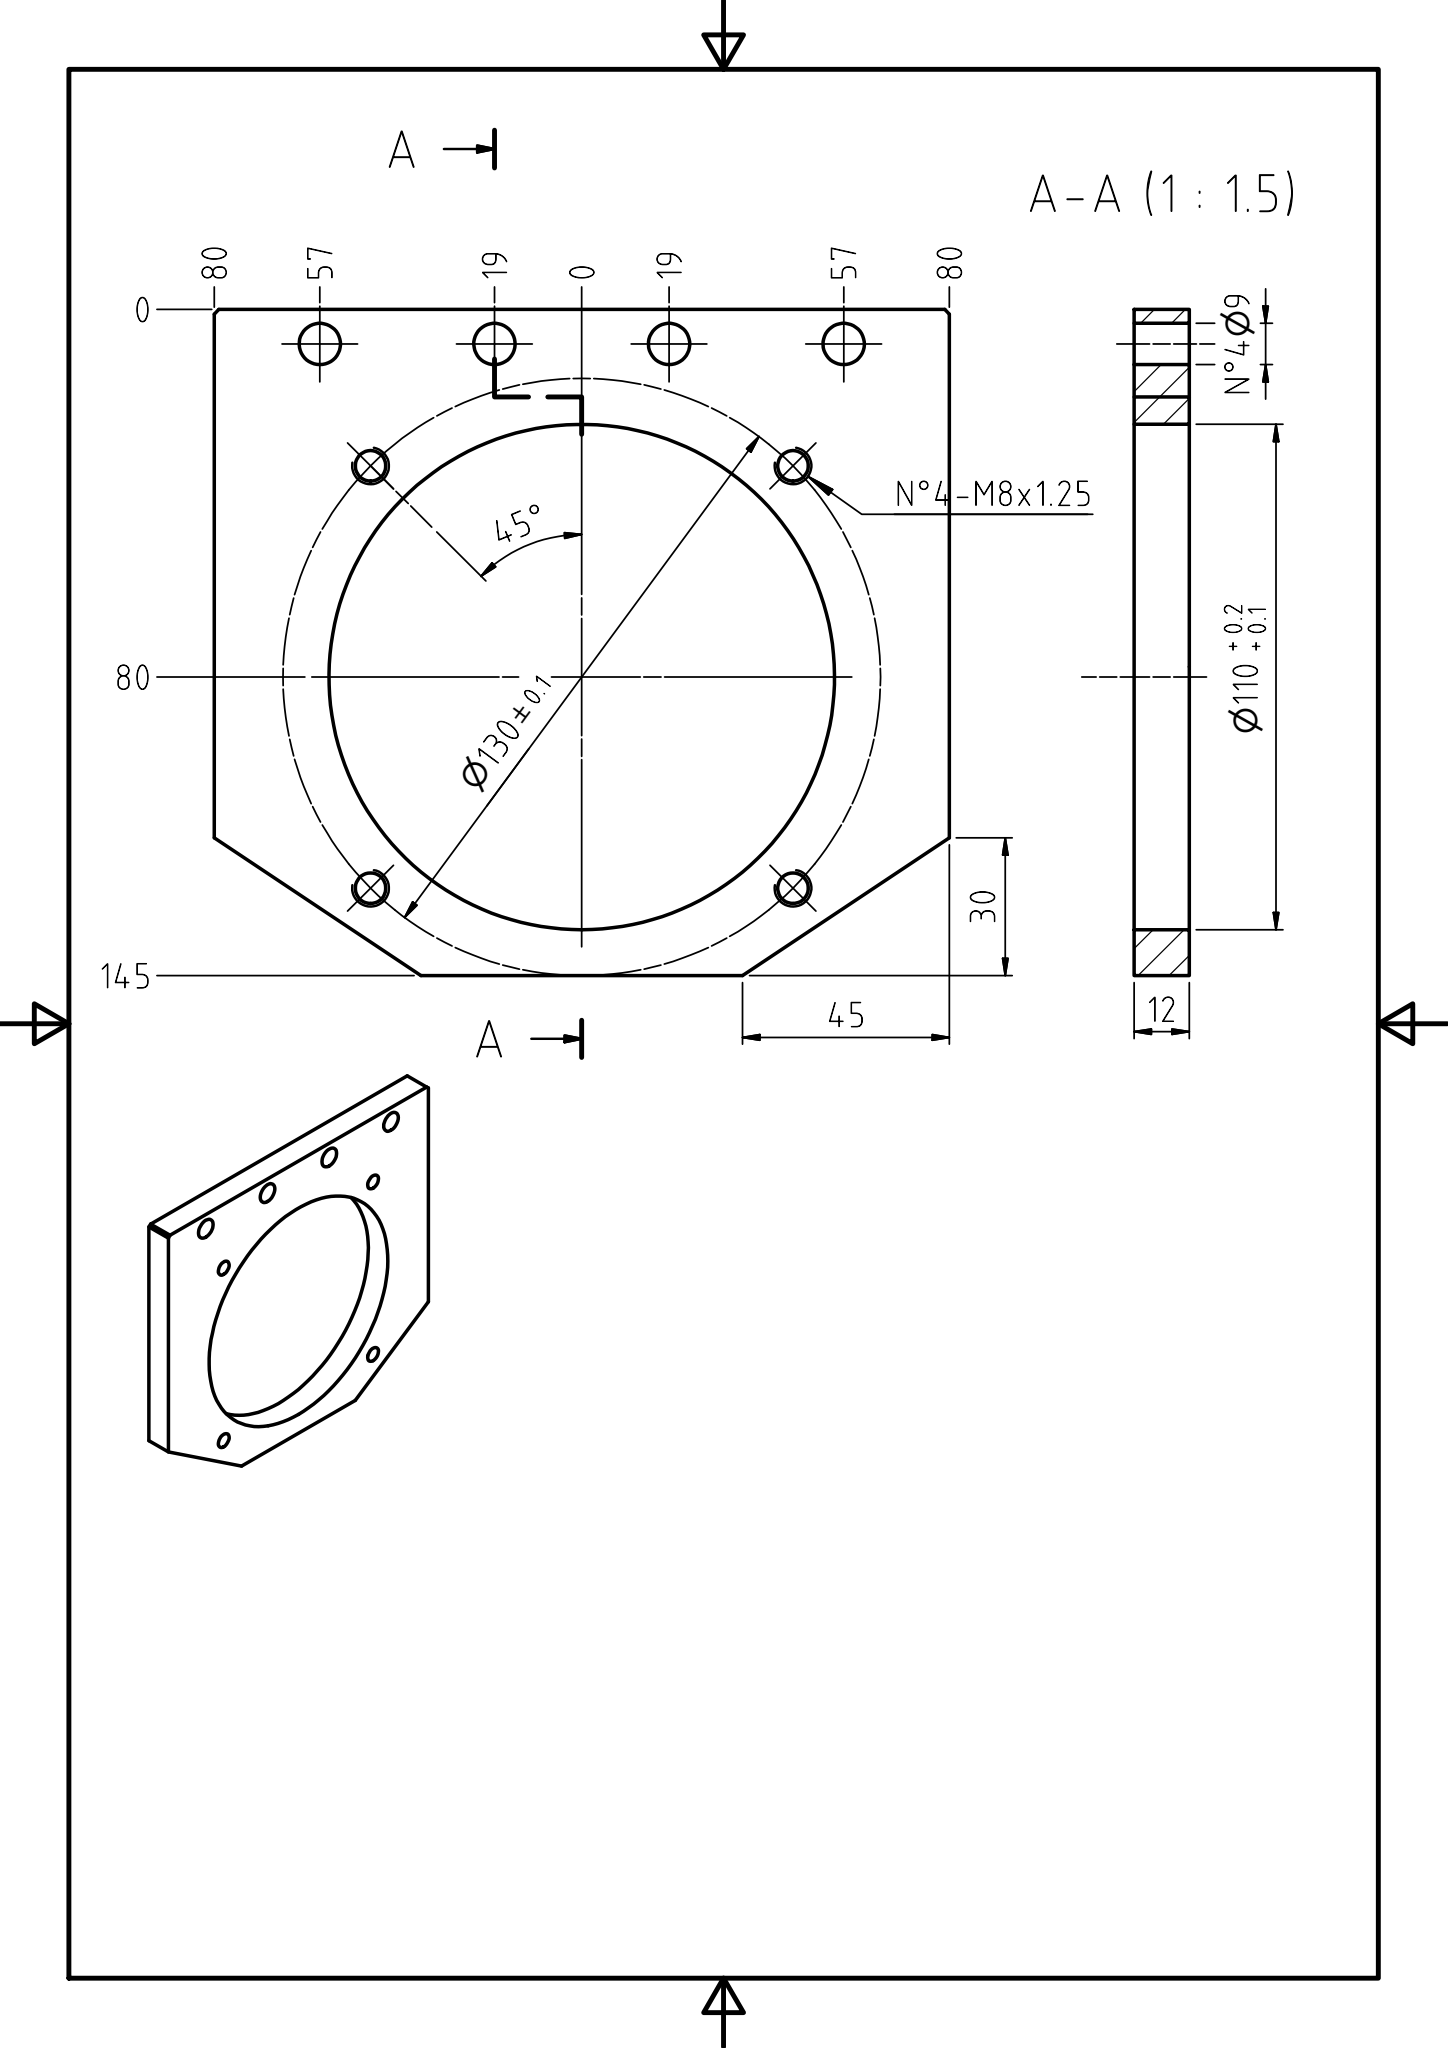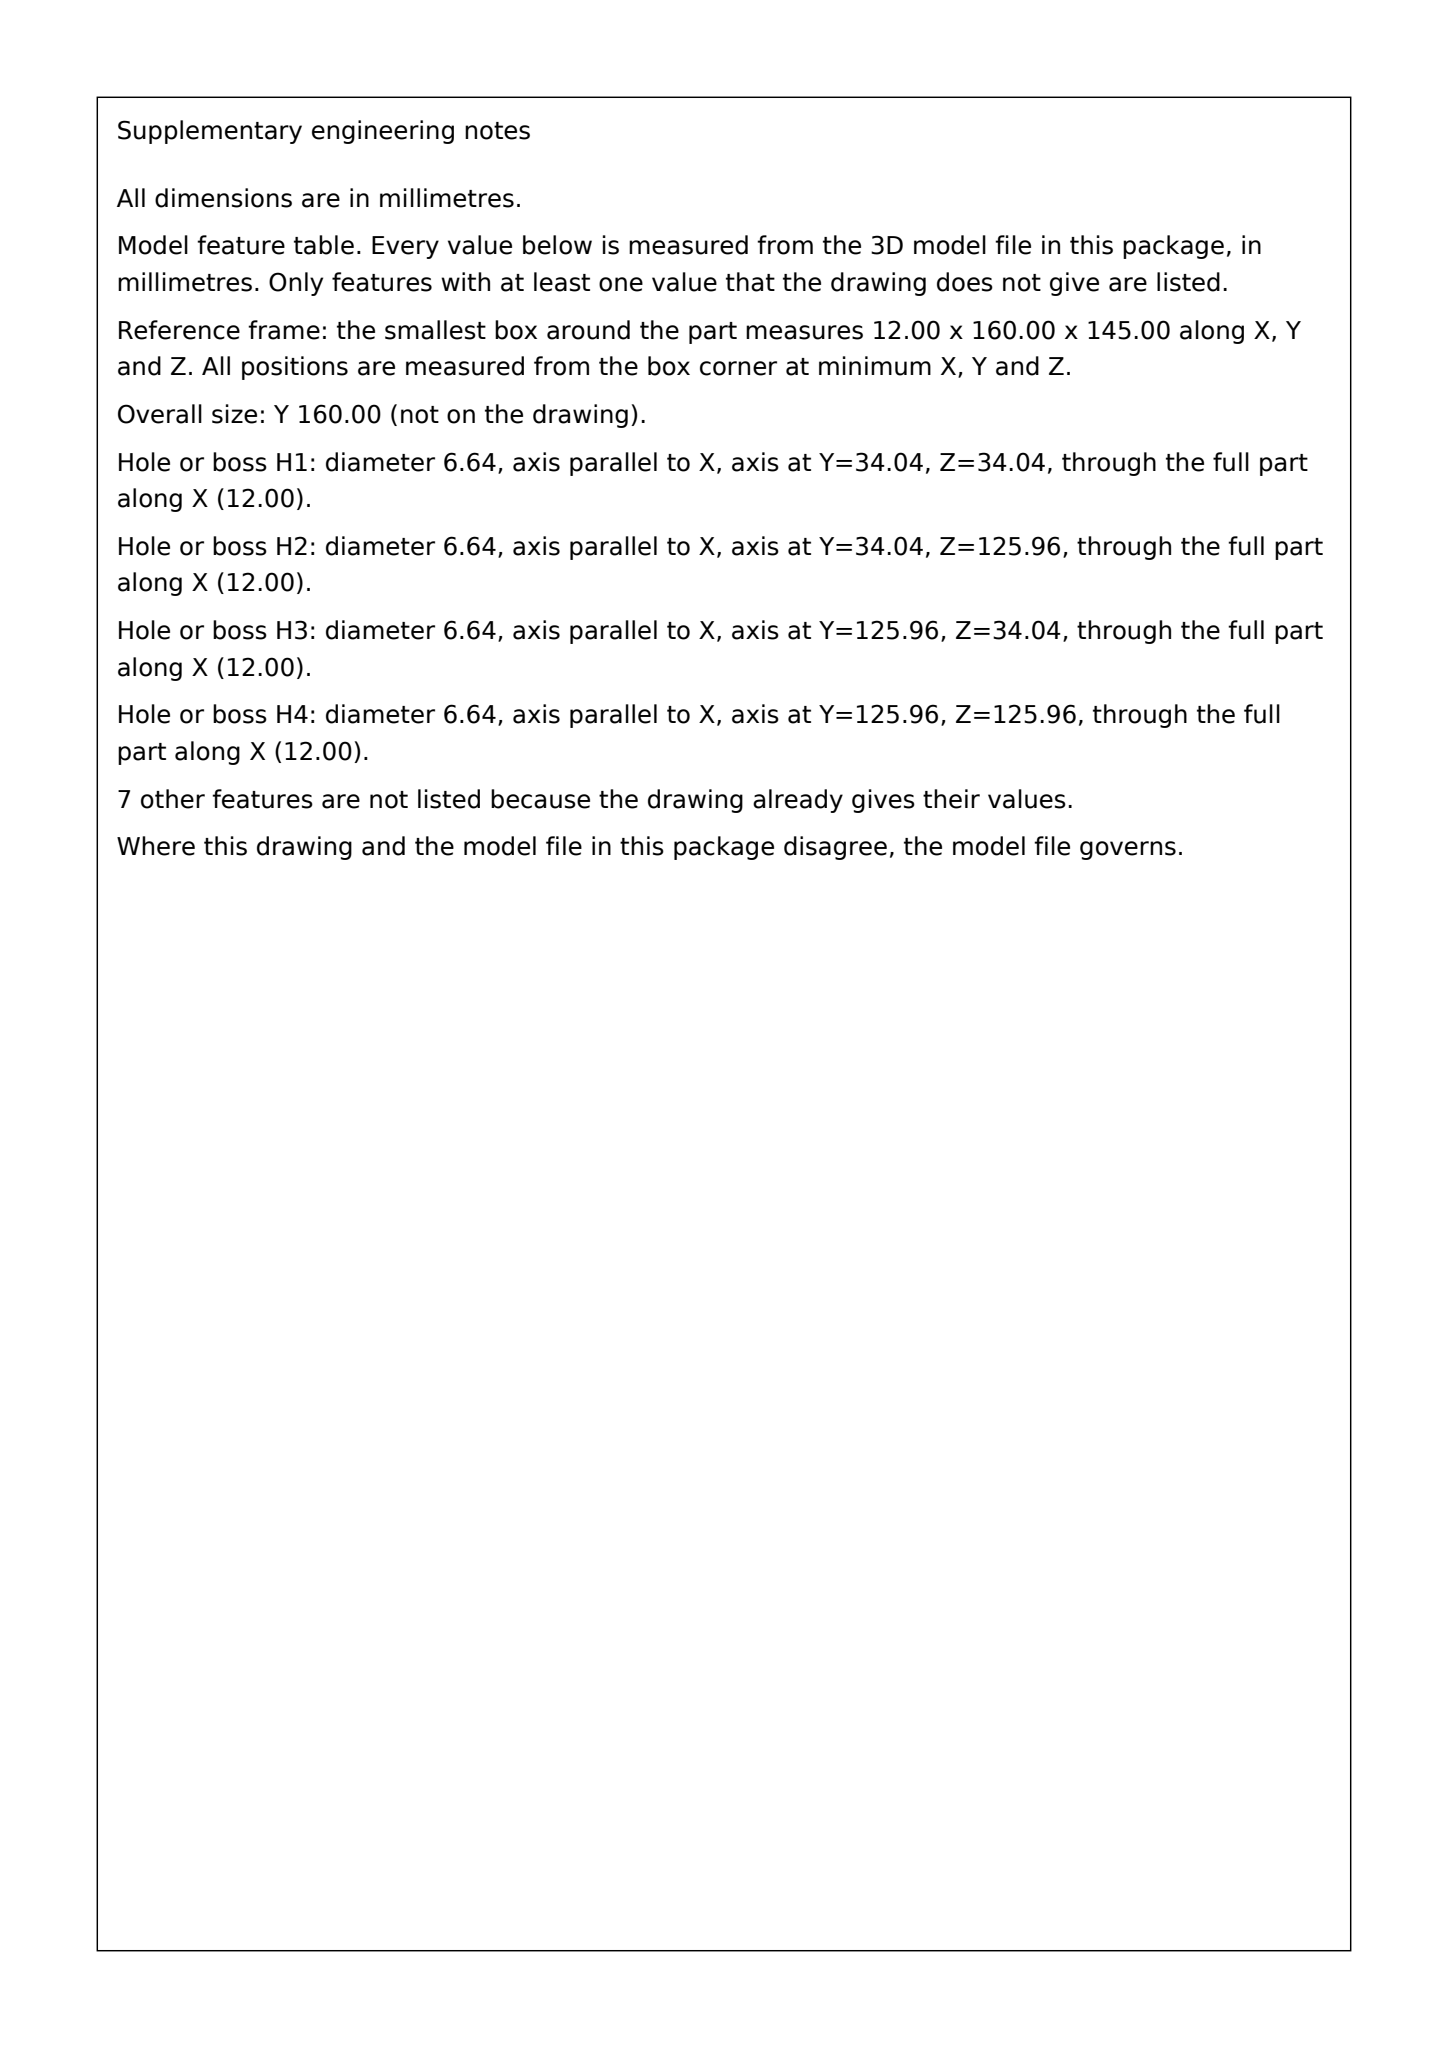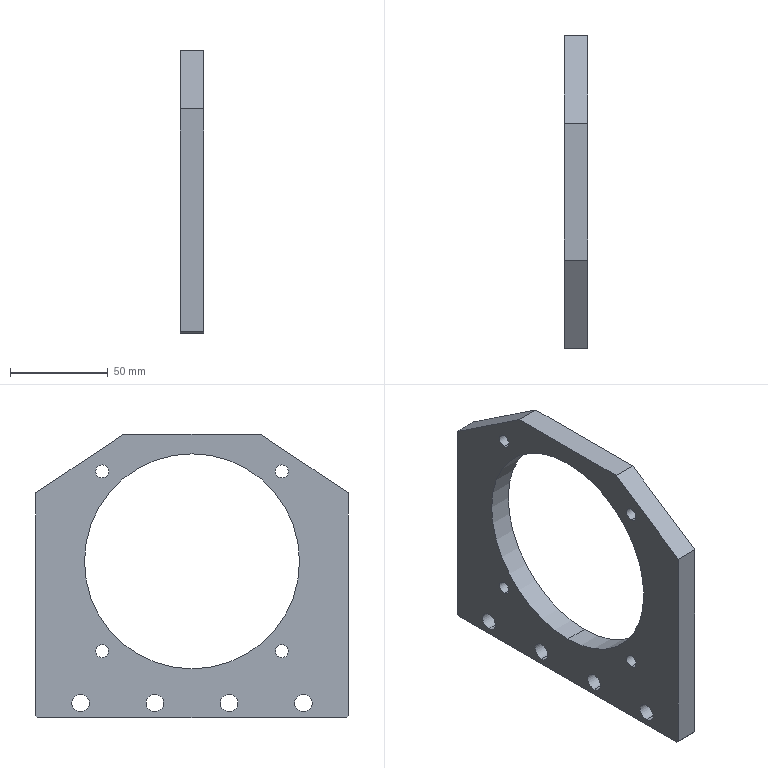Part | SolidWorks | mm | 1 solid | 28 faces | box 12 x 160 x 145 mm | volume 143429 mm3 | cylinder 18 | plane 10 | commonest cylinder face diameters 9 x8 6.647 x8 110 x2